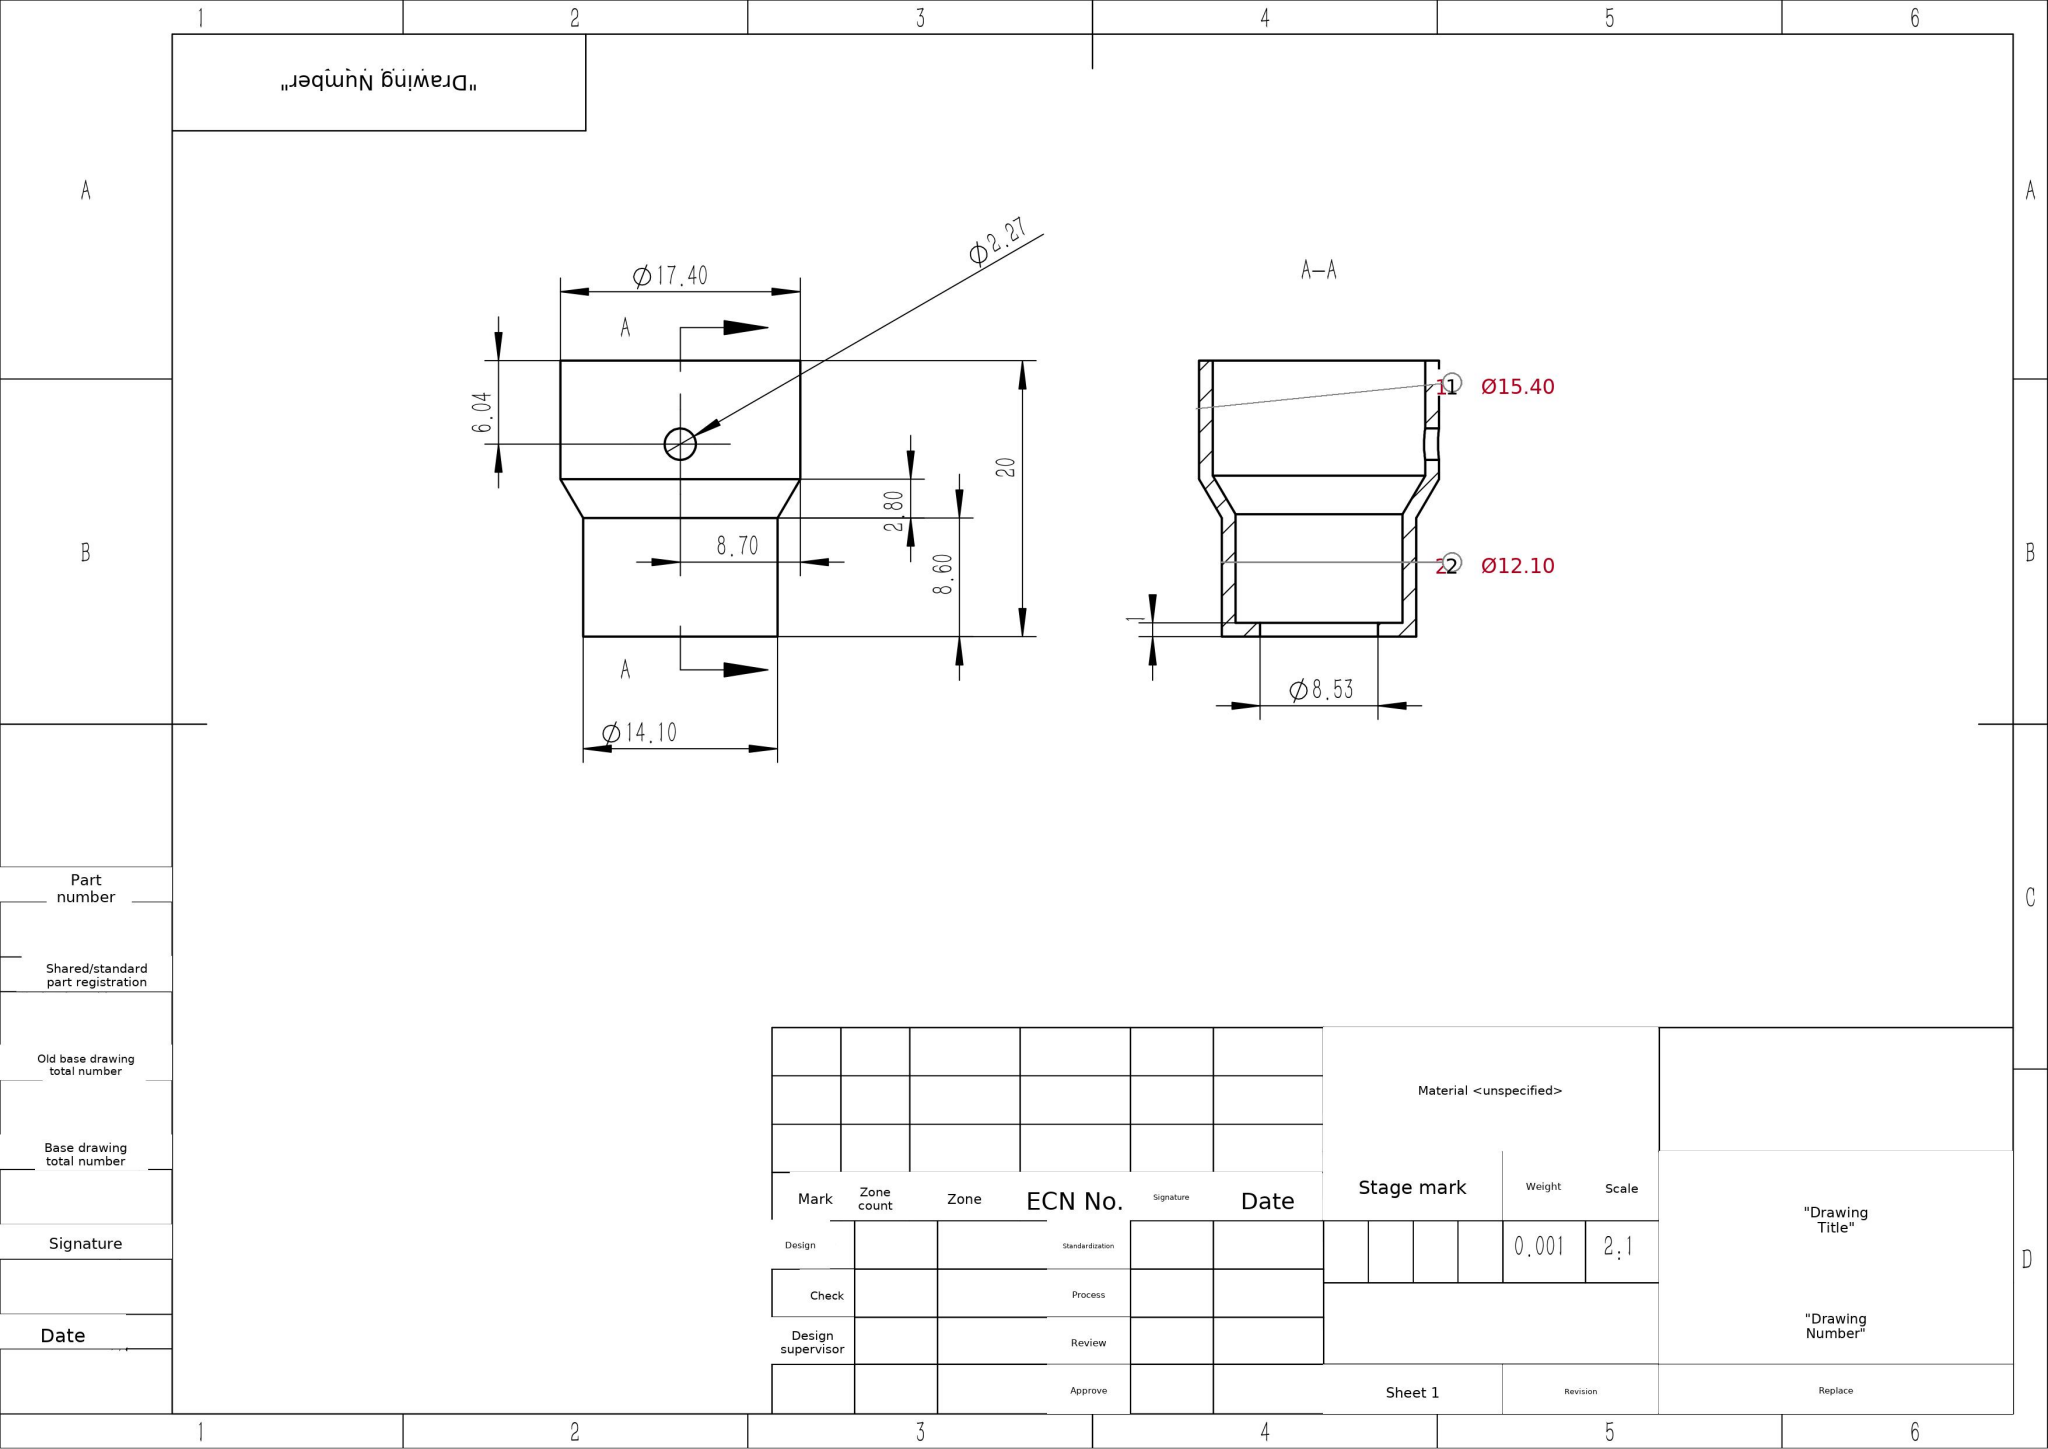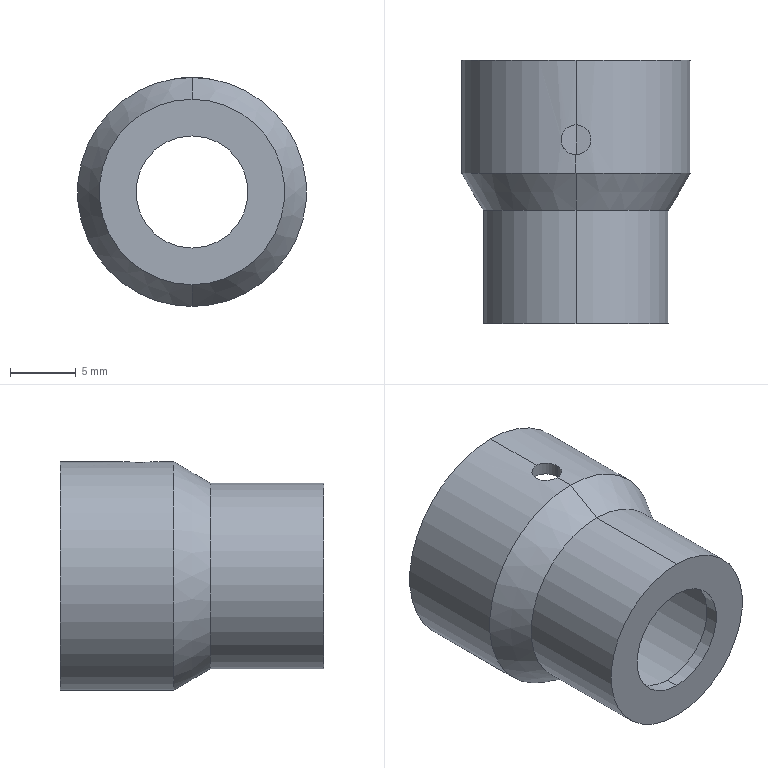Part | SolidWorks | mm | 1 solid | 19 faces | box 17.4 x 20 x 17.4 mm | volume 1000 mm3 | cylinder 12 | cone 4 | plane 3 | commonest cylinder face diameters 2.271 x2 12.1 x2 8.532 x2 14.1 x2 15.402 x2 17.402 x2
build123d program:
from build123d import *

# Parameters (mm, degrees)
SKETCH3_R          = 1.135
CUT_EXTRUDE1_DEPTH = 10


with BuildPart() as part:
    # Sketch1 → Revolve-Thin1 (revolve)
    with BuildSketch(Plane.XY, mode=Mode.PRIVATE) as revolve_thin1_sk:
        Polygon((7.701, 19), (7.701, 10.678), (6.05, 7.876), (6.05, 0), (4.266, 0), (4.266, -1), (7.05, -1), (7.05, 7.603), (8.701, 10.405), (8.701, 19), align=None)
    revolve(revolve_thin1_sk.sketch.rotate(Axis((0, 0, 0), (0, 1, 0)), 90), axis=Axis((0, 0, 0), (0, 1, 0)))

    # Sketch3 → Cut-Extrude1 (cut)
    with BuildSketch(Plane.XY):
        with Locations(Location((0, 12.957, 0), (0, 0, 180))):
            Circle(SKETCH3_R)
    extrude(amount=CUT_EXTRUDE1_DEPTH, mode=Mode.SUBTRACT)


solid = part.part
STEP:
#1=CARTESIAN_POINT('',(1.135,12.957,8.627));
#2=VERTEX_POINT('',#1);
#3=CARTESIAN_POINT('',(-0.,11.821,8.701));
#4=VERTEX_POINT('',#3);
#5=CARTESIAN_POINT('',(1.135,12.957,8.627));
#6=CARTESIAN_POINT('',(1.135,12.808,8.627));
#7=CARTESIAN_POINT('',(1.105,12.659,8.631));
#8=CARTESIAN_POINT('',(0.9922,12.385,8.644));
#9=CARTESIAN_POINT('',(0.9077,12.259,8.654));
#10=CARTESIAN_POINT('',(0.6984,12.049,8.674));
#11=CARTESIAN_POINT('',(0.5726,11.965,8.683));
#12=CARTESIAN_POINT('',(0.2976,11.851,8.697));
#13=CARTESIAN_POINT('',(0.1502,11.821,8.701));
#14=CARTESIAN_POINT('',(-0.,11.821,8.701));
#15=B_SPLINE_CURVE_WITH_KNOTS('',3,(#5,#6,#7,#8,#9,#10,#11,#12,#13,#14),.UNSPECIFIED.,.F.,.F.,(4,2,2,2,4),(0.003553,0.003998,0.004442,0.004886,0.00533),.UNSPECIFIED.);
#16=EDGE_CURVE('',#2,#4,#15,.T.);
#17=ORIENTED_EDGE('',*,*,#16,.F.);
#18=CARTESIAN_POINT('',(1.135,12.957,7.617));
#19=VERTEX_POINT('',#18);
#20=CARTESIAN_POINT('',(1.135,12.957,10.));
#21=DIRECTION('',(0.,0.,-1.));
#22=VECTOR('',#21,1000.);
#23=LINE('',#20,#22);
#24=EDGE_CURVE('',#2,#19,#23,.T.);
#25=ORIENTED_EDGE('',*,*,#24,.T.);
#26=CARTESIAN_POINT('',(0.,11.821,7.701));
#27=VERTEX_POINT('',#26);
#28=CARTESIAN_POINT('',(1.135,12.957,7.617));
#29=CARTESIAN_POINT('',(1.135,12.808,7.617));
#30=CARTESIAN_POINT('',(1.105,12.659,7.621));
#31=CARTESIAN_POINT('',(0.9922,12.385,7.637));
#32=CARTESIAN_POINT('',(0.9077,12.259,7.648));
#33=CARTESIAN_POINT('',(0.6984,12.049,7.67));
#34=CARTESIAN_POINT('',(0.5728,11.965,7.681));
#35=CARTESIAN_POINT('',(0.2976,11.851,7.696));
#36=CARTESIAN_POINT('',(0.1501,11.821,7.701));
#37=CARTESIAN_POINT('',(0.,11.821,7.701));
#38=B_SPLINE_CURVE_WITH_KNOTS('',3,(#28,#29,#30,#31,#32,#33,#34,#35,#36,#37),.UNSPECIFIED.,.F.,.F.,(4,2,2,2,4),(0.003554,0.003999,0.004443,0.004887,0.005332),.UNSPECIFIED.);
#39=EDGE_CURVE('',#19,#27,#38,.T.);
#40=ORIENTED_EDGE('',*,*,#39,.T.);
#41=CARTESIAN_POINT('',(-1.135,12.957,7.617));
#42=VERTEX_POINT('',#41);
#43=CARTESIAN_POINT('',(0.,11.821,7.701));
#44=CARTESIAN_POINT('',(-0.15,11.821,7.701));
#45=CARTESIAN_POINT('',(-0.2975,11.851,7.696));
#46=CARTESIAN_POINT('',(-0.5721,11.965,7.681));
#47=CARTESIAN_POINT('',(-0.698,12.049,7.67));
#48=CARTESIAN_POINT('',(-0.907,12.258,7.648));
#49=CARTESIAN_POINT('',(-0.9916,12.384,7.637));
#50=CARTESIAN_POINT('',(-1.105,12.657,7.622));
#51=CARTESIAN_POINT('',(-1.135,12.806,7.617));
#52=CARTESIAN_POINT('',(-1.135,12.957,7.617));
#53=B_SPLINE_CURVE_WITH_KNOTS('',3,(#43,#44,#45,#46,#47,#48,#49,#50,#51,#52),.UNSPECIFIED.,.F.,.F.,(4,2,2,2,4),(0.005332,0.005776,0.00622,0.006664,0.007108),.UNSPECIFIED.);
#54=EDGE_CURVE('',#27,#42,#53,.T.);
#55=ORIENTED_EDGE('',*,*,#54,.T.);
#56=CARTESIAN_POINT('',(-1.135,12.957,8.627));
#57=VERTEX_POINT('',#56);
#58=CARTESIAN_POINT('',(-1.135,12.957,10.));
#59=DIRECTION('',(0.,0.,-1.));
#60=VECTOR('',#59,1000.);
#61=LINE('',#58,#60);
#62=EDGE_CURVE('',#57,#42,#61,.T.);
#63=ORIENTED_EDGE('',*,*,#62,.F.);
#64=CARTESIAN_POINT('',(-0.,11.821,8.701));
#65=CARTESIAN_POINT('',(-0.15,11.821,8.701));
#66=CARTESIAN_POINT('',(-0.2974,11.851,8.697));
#67=CARTESIAN_POINT('',(-0.5721,11.965,8.683));
#68=CARTESIAN_POINT('',(-0.698,12.049,8.674));
#69=CARTESIAN_POINT('',(-0.9071,12.258,8.654));
#70=CARTESIAN_POINT('',(-0.9917,12.384,8.644));
#71=CARTESIAN_POINT('',(-1.105,12.657,8.631));
#72=CARTESIAN_POINT('',(-1.135,12.807,8.627));
#73=CARTESIAN_POINT('',(-1.135,12.957,8.627));
#74=B_SPLINE_CURVE_WITH_KNOTS('',3,(#64,#65,#66,#67,#68,#69,#70,#71,#72,#73),.UNSPECIFIED.,.F.,.F.,(4,2,2,2,4),(0.00533,0.005774,0.006218,0.006662,0.007106),.UNSPECIFIED.);
#75=EDGE_CURVE('',#4,#57,#74,.T.);
#76=ORIENTED_EDGE('',*,*,#75,.F.);
#77=EDGE_LOOP('',(#17,#25,#40,#55,#63,#76));
#78=FACE_OUTER_BOUND('',#77,.T.);
#79=CARTESIAN_POINT('',(0.,12.957,10.));
#80=DIRECTION('',(0.,0.,-1.));
#81=DIRECTION('',(-1.,0.,0.));
#82=AXIS2_PLACEMENT_3D('',#79,#80,#81);
#83=CYLINDRICAL_SURFACE('',#82,1.135);
#84=ADVANCED_FACE('',(#78),#83,.F.);
#85=CARTESIAN_POINT('',(0.,7.876,6.05));
#86=VERTEX_POINT('',#85);
#87=CARTESIAN_POINT('',(0.,7.876,-6.05));
#88=VERTEX_POINT('',#87);
#89=CARTESIAN_POINT('',(0.,7.876,0.));
#90=DIRECTION('',(0.,-1.,0.));
#91=DIRECTION('',(0.,0.,-1.));
#92=AXIS2_PLACEMENT_3D('',#89,#90,#91);
#93=CIRCLE('',#92,6.05);
#94=EDGE_CURVE('',#86,#88,#93,.T.);
#95=ORIENTED_EDGE('',*,*,#94,.T.);
#96=CARTESIAN_POINT('',(0.,10.678,-7.701));
#97=VERTEX_POINT('',#96);
#98=CARTESIAN_POINT('',(0.,7.876,-6.05));
#99=DIRECTION('',(0.,0.8616,-0.5076));
#100=VECTOR('',#99,1000.);
#101=LINE('',#98,#100);
#102=EDGE_CURVE('',#88,#97,#101,.T.);
#103=ORIENTED_EDGE('',*,*,#102,.T.);
#104=CARTESIAN_POINT('',(0.,10.678,7.701));
#105=VERTEX_POINT('',#104);
#106=CARTESIAN_POINT('',(0.,10.678,0.));
#107=DIRECTION('',(0.,-1.,0.));
#108=DIRECTION('',(0.,0.,-1.));
#109=AXIS2_PLACEMENT_3D('',#106,#107,#108);
#110=CIRCLE('',#109,7.701);
#111=EDGE_CURVE('',#105,#97,#110,.T.);
#112=ORIENTED_EDGE('',*,*,#111,.F.);
#113=CARTESIAN_POINT('',(0.,7.876,6.05));
#114=DIRECTION('',(0.,0.8616,0.5076));
#115=VECTOR('',#114,1000.);
#116=LINE('',#113,#115);
#117=EDGE_CURVE('',#86,#105,#116,.T.);
#118=ORIENTED_EDGE('',*,*,#117,.F.);
#119=EDGE_LOOP('',(#95,#103,#112,#118));
#120=FACE_OUTER_BOUND('',#119,.T.);
#121=CARTESIAN_POINT('',(0.,7.876,0.));
#122=DIRECTION('',(0.,1.,0.));
#123=DIRECTION('',(0.,0.,1.));
#124=AXIS2_PLACEMENT_3D('',#121,#122,#123);
#125=CONICAL_SURFACE('',#124,6.05,0.5324);
#126=ADVANCED_FACE('',(#120),#125,.F.);
#127=ORIENTED_EDGE('',*,*,#94,.F.);
#128=CARTESIAN_POINT('',(0.,0.,6.05));
#129=VERTEX_POINT('',#128);
#130=CARTESIAN_POINT('',(0.,0.,6.05));
#131=DIRECTION('',(0.,-1.,0.));
#132=VECTOR('',#131,1000.);
#133=LINE('',#130,#132);
#134=EDGE_CURVE('',#86,#129,#133,.T.);
#135=ORIENTED_EDGE('',*,*,#134,.T.);
#136=CARTESIAN_POINT('',(0.,0.,-6.05));
#137=VERTEX_POINT('',#136);
#138=CARTESIAN_POINT('',(0.,0.,0.));
#139=DIRECTION('',(0.,-1.,0.));
#140=DIRECTION('',(0.,0.,-1.));
#141=AXIS2_PLACEMENT_3D('',#138,#139,#140);
#142=CIRCLE('',#141,6.05);
#143=EDGE_CURVE('',#129,#137,#142,.T.);
#144=ORIENTED_EDGE('',*,*,#143,.T.);
#145=CARTESIAN_POINT('',(0.,0.,-6.05));
#146=DIRECTION('',(0.,-1.,0.));
#147=VECTOR('',#146,1000.);
#148=LINE('',#145,#147);
#149=EDGE_CURVE('',#88,#137,#148,.T.);
#150=ORIENTED_EDGE('',*,*,#149,.F.);
#151=EDGE_LOOP('',(#127,#135,#144,#150));
#152=FACE_OUTER_BOUND('',#151,.T.);
#153=CARTESIAN_POINT('',(0.,0.,0.));
#154=DIRECTION('',(0.,-1.,0.));
#155=DIRECTION('',(0.,0.,-1.));
#156=AXIS2_PLACEMENT_3D('',#153,#154,#155);
#157=CYLINDRICAL_SURFACE('',#156,6.05);
#158=ADVANCED_FACE('',(#152),#157,.F.);
#159=CARTESIAN_POINT('',(0.,0.,4.266));
#160=VERTEX_POINT('',#159);
#161=CARTESIAN_POINT('',(0.,0.,-4.266));
#162=VERTEX_POINT('',#161);
#163=CARTESIAN_POINT('',(0.,0.,0.));
#164=DIRECTION('',(0.,-1.,0.));
#165=DIRECTION('',(0.,0.,-1.));
#166=AXIS2_PLACEMENT_3D('',#163,#164,#165);
#167=CIRCLE('',#166,4.266);
#168=EDGE_CURVE('',#160,#162,#167,.T.);
#169=ORIENTED_EDGE('',*,*,#168,.F.);
#170=CARTESIAN_POINT('',(0.,-1.,4.266));
#171=VERTEX_POINT('',#170);
#172=CARTESIAN_POINT('',(0.,0.,4.266));
#173=DIRECTION('',(0.,-1.,0.));
#174=VECTOR('',#173,1000.);
#175=LINE('',#172,#174);
#176=EDGE_CURVE('',#160,#171,#175,.T.);
#177=ORIENTED_EDGE('',*,*,#176,.T.);
#178=CARTESIAN_POINT('',(0.,-1.,-4.266));
#179=VERTEX_POINT('',#178);
#180=CARTESIAN_POINT('',(0.,-1.,0.));
#181=DIRECTION('',(0.,-1.,0.));
#182=DIRECTION('',(0.,0.,-1.));
#183=AXIS2_PLACEMENT_3D('',#180,#181,#182);
#184=CIRCLE('',#183,4.266);
#185=EDGE_CURVE('',#171,#179,#184,.T.);
#186=ORIENTED_EDGE('',*,*,#185,.T.);
#187=CARTESIAN_POINT('',(0.,0.,-4.266));
#188=DIRECTION('',(0.,-1.,0.));
#189=VECTOR('',#188,1000.);
#190=LINE('',#187,#189);
#191=EDGE_CURVE('',#162,#179,#190,.T.);
#192=ORIENTED_EDGE('',*,*,#191,.F.);
#193=EDGE_LOOP('',(#169,#177,#186,#192));
#194=FACE_OUTER_BOUND('',#193,.T.);
#195=CARTESIAN_POINT('',(0.,0.,0.));
#196=DIRECTION('',(0.,-1.,0.));
#197=DIRECTION('',(0.,0.,-1.));
#198=AXIS2_PLACEMENT_3D('',#195,#196,#197);
#199=CYLINDRICAL_SURFACE('',#198,4.266);
#200=ADVANCED_FACE('',(#194),#199,.F.);
#201=CARTESIAN_POINT('',(0.,7.603,-7.05));
#202=VERTEX_POINT('',#201);
#203=CARTESIAN_POINT('',(0.,7.603,7.05));
#204=VERTEX_POINT('',#203);
#205=CARTESIAN_POINT('',(0.,7.603,0.));
#206=DIRECTION('',(0.,-1.,0.));
#207=DIRECTION('',(0.,0.,-1.));
#208=AXIS2_PLACEMENT_3D('',#205,#206,#207);
#209=CIRCLE('',#208,7.05);
#210=EDGE_CURVE('',#202,#204,#209,.T.);
#211=ORIENTED_EDGE('',*,*,#210,.T.);
#212=CARTESIAN_POINT('',(0.,-1.,7.05));
#213=VERTEX_POINT('',#212);
#214=CARTESIAN_POINT('',(0.,0.,7.05));
#215=DIRECTION('',(0.,-1.,0.));
#216=VECTOR('',#215,1000.);
#217=LINE('',#214,#216);
#218=EDGE_CURVE('',#204,#213,#217,.T.);
#219=ORIENTED_EDGE('',*,*,#218,.T.);
#220=CARTESIAN_POINT('',(0.,-1.,-7.05));
#221=VERTEX_POINT('',#220);
#222=CARTESIAN_POINT('',(0.,-1.,0.));
#223=DIRECTION('',(0.,-1.,0.));
#224=DIRECTION('',(0.,0.,-1.));
#225=AXIS2_PLACEMENT_3D('',#222,#223,#224);
#226=CIRCLE('',#225,7.05);
#227=EDGE_CURVE('',#221,#213,#226,.T.);
#228=ORIENTED_EDGE('',*,*,#227,.F.);
#229=CARTESIAN_POINT('',(0.,0.,-7.05));
#230=DIRECTION('',(0.,-1.,0.));
#231=VECTOR('',#230,1000.);
#232=LINE('',#229,#231);
#233=EDGE_CURVE('',#202,#221,#232,.T.);
#234=ORIENTED_EDGE('',*,*,#233,.F.);
#235=EDGE_LOOP('',(#211,#219,#228,#234));
#236=FACE_OUTER_BOUND('',#235,.T.);
#237=CARTESIAN_POINT('',(0.,0.,0.));
#238=DIRECTION('',(0.,-1.,0.));
#239=DIRECTION('',(0.,0.,-1.));
#240=AXIS2_PLACEMENT_3D('',#237,#238,#239);
#241=CYLINDRICAL_SURFACE('',#240,7.05);
#242=ADVANCED_FACE('',(#236),#241,.T.);
#243=ORIENTED_EDGE('',*,*,#210,.F.);
#244=CARTESIAN_POINT('',(0.,10.405,-8.701));
#245=VERTEX_POINT('',#244);
#246=CARTESIAN_POINT('',(0.,7.603,-7.05));
#247=DIRECTION('',(0.,0.8616,-0.5076));
#248=VECTOR('',#247,1000.);
#249=LINE('',#246,#248);
#250=EDGE_CURVE('',#202,#245,#249,.T.);
#251=ORIENTED_EDGE('',*,*,#250,.T.);
#252=CARTESIAN_POINT('',(0.,10.405,8.701));
#253=VERTEX_POINT('',#252);
#254=CARTESIAN_POINT('',(0.,10.405,0.));
#255=DIRECTION('',(0.,-1.,0.));
#256=DIRECTION('',(0.,0.,-1.));
#257=AXIS2_PLACEMENT_3D('',#254,#255,#256);
#258=CIRCLE('',#257,8.701);
#259=EDGE_CURVE('',#245,#253,#258,.T.);
#260=ORIENTED_EDGE('',*,*,#259,.T.);
#261=CARTESIAN_POINT('',(0.,7.603,7.05));
#262=DIRECTION('',(0.,0.8616,0.5076));
#263=VECTOR('',#262,1000.);
#264=LINE('',#261,#263);
#265=EDGE_CURVE('',#204,#253,#264,.T.);
#266=ORIENTED_EDGE('',*,*,#265,.F.);
#267=EDGE_LOOP('',(#243,#251,#260,#266));
#268=FACE_OUTER_BOUND('',#267,.T.);
#269=CARTESIAN_POINT('',(0.,7.603,0.));
#270=DIRECTION('',(0.,1.,0.));
#271=DIRECTION('',(0.,0.,1.));
#272=AXIS2_PLACEMENT_3D('',#269,#270,#271);
#273=CONICAL_SURFACE('',#272,7.05,0.5324);
#274=ADVANCED_FACE('',(#268),#273,.T.);
#275=CARTESIAN_POINT('',(0.,19.,7.701));
#276=VERTEX_POINT('',#275);
#277=CARTESIAN_POINT('',(0.,19.,-7.701));
#278=VERTEX_POINT('',#277);
#279=CARTESIAN_POINT('',(0.,19.,0.));
#280=DIRECTION('',(0.,-1.,0.));
#281=DIRECTION('',(0.,0.,-1.));
#282=AXIS2_PLACEMENT_3D('',#279,#280,#281);
#283=CIRCLE('',#282,7.701);
#284=EDGE_CURVE('',#276,#278,#283,.T.);
#285=ORIENTED_EDGE('',*,*,#284,.F.);
#286=CARTESIAN_POINT('',(0.,14.092,7.701));
#287=VERTEX_POINT('',#286);
#288=CARTESIAN_POINT('',(0.,0.,7.701));
#289=DIRECTION('',(0.,-1.,0.));
#290=VECTOR('',#289,1000.);
#291=LINE('',#288,#290);
#292=EDGE_CURVE('',#276,#287,#291,.T.);
#293=ORIENTED_EDGE('',*,*,#292,.T.);
#294=CARTESIAN_POINT('',(-1.135,12.957,7.617));
#295=CARTESIAN_POINT('',(-1.135,13.107,7.617));
#296=CARTESIAN_POINT('',(-1.106,13.254,7.621));
#297=CARTESIAN_POINT('',(-0.9915,13.529,7.637));
#298=CARTESIAN_POINT('',(-0.9071,13.655,7.648));
#299=CARTESIAN_POINT('',(-0.6978,13.864,7.67));
#300=CARTESIAN_POINT('',(-0.5712,13.949,7.681));
#301=CARTESIAN_POINT('',(-0.298,14.062,7.696));
#302=CARTESIAN_POINT('',(-0.1484,14.092,7.701));
#303=CARTESIAN_POINT('',(0.,14.092,7.701));
#304=B_SPLINE_CURVE_WITH_KNOTS('',3,(#294,#295,#296,#297,#298,#299,#300,#301,#302,#303),.UNSPECIFIED.,.F.,.F.,(4,2,2,2,4),(0.,0.0004444,0.0008888,0.001333,0.001778),.UNSPECIFIED.);
#305=EDGE_CURVE('',#42,#287,#304,.T.);
#306=ORIENTED_EDGE('',*,*,#305,.F.);
#307=ORIENTED_EDGE('',*,*,#54,.F.);
#308=CARTESIAN_POINT('',(0.,0.,7.701));
#309=DIRECTION('',(0.,-1.,0.));
#310=VECTOR('',#309,1000.);
#311=LINE('',#308,#310);
#312=EDGE_CURVE('',#27,#105,#311,.T.);
#313=ORIENTED_EDGE('',*,*,#312,.T.);
#314=ORIENTED_EDGE('',*,*,#111,.T.);
#315=CARTESIAN_POINT('',(0.,0.,-7.701));
#316=DIRECTION('',(0.,-1.,0.));
#317=VECTOR('',#316,1000.);
#318=LINE('',#315,#317);
#319=EDGE_CURVE('',#278,#97,#318,.T.);
#320=ORIENTED_EDGE('',*,*,#319,.F.);
#321=EDGE_LOOP('',(#285,#293,#306,#307,#313,#314,#320));
#322=FACE_OUTER_BOUND('',#321,.T.);
#323=CARTESIAN_POINT('',(0.,0.,0.));
#324=DIRECTION('',(0.,-1.,0.));
#325=DIRECTION('',(0.,0.,-1.));
#326=AXIS2_PLACEMENT_3D('',#323,#324,#325);
#327=CYLINDRICAL_SURFACE('',#326,7.701);
#328=ADVANCED_FACE('',(#322),#327,.F.);
#329=CARTESIAN_POINT('',(0.,19.,-8.701));
#330=VERTEX_POINT('',#329);
#331=CARTESIAN_POINT('',(0.,19.,8.701));
#332=VERTEX_POINT('',#331);
#333=CARTESIAN_POINT('',(0.,19.,0.));
#334=DIRECTION('',(0.,-1.,0.));
#335=DIRECTION('',(0.,0.,-1.));
#336=AXIS2_PLACEMENT_3D('',#333,#334,#335);
#337=CIRCLE('',#336,8.701);
#338=EDGE_CURVE('',#330,#332,#337,.T.);
#339=ORIENTED_EDGE('',*,*,#338,.T.);
#340=CARTESIAN_POINT('',(0.,14.092,8.701));
#341=VERTEX_POINT('',#340);
#342=CARTESIAN_POINT('',(0.,0.,8.701));
#343=DIRECTION('',(0.,-1.,0.));
#344=VECTOR('',#343,1000.);
#345=LINE('',#342,#344);
#346=EDGE_CURVE('',#332,#341,#345,.T.);
#347=ORIENTED_EDGE('',*,*,#346,.T.);
#348=CARTESIAN_POINT('',(0.,14.092,8.701));
#349=CARTESIAN_POINT('',(0.1482,14.092,8.701));
#350=CARTESIAN_POINT('',(0.2971,14.062,8.697));
#351=CARTESIAN_POINT('',(0.5721,13.948,8.683));
#352=CARTESIAN_POINT('',(0.697,13.865,8.674));
#353=CARTESIAN_POINT('',(0.9087,13.653,8.654));
#354=CARTESIAN_POINT('',(0.992,13.529,8.644));
#355=CARTESIAN_POINT('',(1.106,13.254,8.631));
#356=CARTESIAN_POINT('',(1.135,13.105,8.627));
#357=CARTESIAN_POINT('',(1.135,12.957,8.627));
#358=B_SPLINE_CURVE_WITH_KNOTS('',3,(#348,#349,#350,#351,#352,#353,#354,#355,#356,#357),.UNSPECIFIED.,.F.,.F.,(4,2,2,2,4),(0.001777,0.002221,0.002665,0.003109,0.003553),.UNSPECIFIED.);
#359=EDGE_CURVE('',#341,#2,#358,.T.);
#360=ORIENTED_EDGE('',*,*,#359,.T.);
#361=ORIENTED_EDGE('',*,*,#16,.T.);
#362=CARTESIAN_POINT('',(0.,0.,8.701));
#363=DIRECTION('',(0.,-1.,0.));
#364=VECTOR('',#363,1000.);
#365=LINE('',#362,#364);
#366=EDGE_CURVE('',#4,#253,#365,.T.);
#367=ORIENTED_EDGE('',*,*,#366,.T.);
#368=ORIENTED_EDGE('',*,*,#259,.F.);
#369=CARTESIAN_POINT('',(0.,0.,-8.701));
#370=DIRECTION('',(0.,-1.,0.));
#371=VECTOR('',#370,1000.);
#372=LINE('',#369,#371);
#373=EDGE_CURVE('',#330,#245,#372,.T.);
#374=ORIENTED_EDGE('',*,*,#373,.F.);
#375=EDGE_LOOP('',(#339,#347,#360,#361,#367,#368,#374));
#376=FACE_OUTER_BOUND('',#375,.T.);
#377=CARTESIAN_POINT('',(0.,0.,0.));
#378=DIRECTION('',(0.,-1.,0.));
#379=DIRECTION('',(0.,0.,-1.));
#380=AXIS2_PLACEMENT_3D('',#377,#378,#379);
#381=CYLINDRICAL_SURFACE('',#380,8.701);
#382=ADVANCED_FACE('',(#376),#381,.T.);
#383=ORIENTED_EDGE('',*,*,#346,.F.);
#384=CARTESIAN_POINT('',(0.,19.,0.));
#385=DIRECTION('',(0.,-1.,0.));
#386=DIRECTION('',(0.,0.,-1.));
#387=AXIS2_PLACEMENT_3D('',#384,#385,#386);
#388=CIRCLE('',#387,8.701);
#389=EDGE_CURVE('',#332,#330,#388,.T.);
#390=ORIENTED_EDGE('',*,*,#389,.T.);
#391=ORIENTED_EDGE('',*,*,#373,.T.);
#392=CARTESIAN_POINT('',(0.,10.405,0.));
#393=DIRECTION('',(0.,-1.,0.));
#394=DIRECTION('',(0.,0.,-1.));
#395=AXIS2_PLACEMENT_3D('',#392,#393,#394);
#396=CIRCLE('',#395,8.701);
#397=EDGE_CURVE('',#253,#245,#396,.T.);
#398=ORIENTED_EDGE('',*,*,#397,.F.);
#399=ORIENTED_EDGE('',*,*,#366,.F.);
#400=ORIENTED_EDGE('',*,*,#75,.T.);
#401=CARTESIAN_POINT('',(-1.135,12.957,8.627));
#402=CARTESIAN_POINT('',(-1.135,13.107,8.627));
#403=CARTESIAN_POINT('',(-1.106,13.254,8.631));
#404=CARTESIAN_POINT('',(-0.9916,13.529,8.644));
#405=CARTESIAN_POINT('',(-0.9072,13.655,8.654));
#406=CARTESIAN_POINT('',(-0.6978,13.864,8.674));
#407=CARTESIAN_POINT('',(-0.5712,13.949,8.683));
#408=CARTESIAN_POINT('',(-0.2979,14.062,8.697));
#409=CARTESIAN_POINT('',(-0.1483,14.092,8.701));
#410=CARTESIAN_POINT('',(0.,14.092,8.701));
#411=B_SPLINE_CURVE_WITH_KNOTS('',3,(#401,#402,#403,#404,#405,#406,#407,#408,#409,#410),.UNSPECIFIED.,.F.,.F.,(4,2,2,2,4),(0.,0.0004443,0.0008885,0.001333,0.001777),.UNSPECIFIED.);
#412=EDGE_CURVE('',#57,#341,#411,.T.);
#413=ORIENTED_EDGE('',*,*,#412,.T.);
#414=EDGE_LOOP('',(#383,#390,#391,#398,#399,#400,#413));
#415=FACE_OUTER_BOUND('',#414,.T.);
#416=CARTESIAN_POINT('',(0.,0.,0.));
#417=DIRECTION('',(0.,-1.,0.));
#418=DIRECTION('',(0.,0.,-1.));
#419=AXIS2_PLACEMENT_3D('',#416,#417,#418);
#420=CYLINDRICAL_SURFACE('',#419,8.701);
#421=ADVANCED_FACE('',(#415),#420,.T.);
#422=ORIENTED_EDGE('',*,*,#292,.F.);
#423=CARTESIAN_POINT('',(0.,19.,0.));
#424=DIRECTION('',(0.,-1.,0.));
#425=DIRECTION('',(0.,0.,-1.));
#426=AXIS2_PLACEMENT_3D('',#423,#424,#425);
#427=CIRCLE('',#426,7.701);
#428=EDGE_CURVE('',#278,#276,#427,.T.);
#429=ORIENTED_EDGE('',*,*,#428,.F.);
#430=ORIENTED_EDGE('',*,*,#319,.T.);
#431=CARTESIAN_POINT('',(0.,10.678,0.));
#432=DIRECTION('',(0.,-1.,0.));
#433=DIRECTION('',(0.,0.,-1.));
#434=AXIS2_PLACEMENT_3D('',#431,#432,#433);
#435=CIRCLE('',#434,7.701);
#436=EDGE_CURVE('',#97,#105,#435,.T.);
#437=ORIENTED_EDGE('',*,*,#436,.T.);
#438=ORIENTED_EDGE('',*,*,#312,.F.);
#439=ORIENTED_EDGE('',*,*,#39,.F.);
#440=CARTESIAN_POINT('',(0.,14.092,7.701));
#441=CARTESIAN_POINT('',(0.1483,14.092,7.701));
#442=CARTESIAN_POINT('',(0.2971,14.062,7.696));
#443=CARTESIAN_POINT('',(0.5722,13.948,7.681));
#444=CARTESIAN_POINT('',(0.6971,13.865,7.67));
#445=CARTESIAN_POINT('',(0.9087,13.653,7.648));
#446=CARTESIAN_POINT('',(0.9919,13.529,7.637));
#447=CARTESIAN_POINT('',(1.106,13.254,7.621));
#448=CARTESIAN_POINT('',(1.135,13.105,7.617));
#449=CARTESIAN_POINT('',(1.135,12.957,7.617));
#450=B_SPLINE_CURVE_WITH_KNOTS('',3,(#440,#441,#442,#443,#444,#445,#446,#447,#448,#449),.UNSPECIFIED.,.F.,.F.,(4,2,2,2,4),(0.001778,0.002222,0.002666,0.00311,0.003554),.UNSPECIFIED.);
#451=EDGE_CURVE('',#287,#19,#450,.T.);
#452=ORIENTED_EDGE('',*,*,#451,.F.);
#453=EDGE_LOOP('',(#422,#429,#430,#437,#438,#439,#452));
#454=FACE_OUTER_BOUND('',#453,.T.);
#455=CARTESIAN_POINT('',(0.,0.,0.));
#456=DIRECTION('',(0.,-1.,0.));
#457=DIRECTION('',(0.,0.,-1.));
#458=AXIS2_PLACEMENT_3D('',#455,#456,#457);
#459=CYLINDRICAL_SURFACE('',#458,7.701);
#460=ADVANCED_FACE('',(#454),#459,.F.);
#461=ORIENTED_EDGE('',*,*,#250,.F.);
#462=CARTESIAN_POINT('',(0.,7.603,0.));
#463=DIRECTION('',(0.,-1.,0.));
#464=DIRECTION('',(0.,0.,-1.));
#465=AXIS2_PLACEMENT_3D('',#462,#463,#464);
#466=CIRCLE('',#465,7.05);
#467=EDGE_CURVE('',#204,#202,#466,.T.);
#468=ORIENTED_EDGE('',*,*,#467,.F.);
#469=ORIENTED_EDGE('',*,*,#265,.T.);
#470=ORIENTED_EDGE('',*,*,#397,.T.);
#471=EDGE_LOOP('',(#461,#468,#469,#470));
#472=FACE_OUTER_BOUND('',#471,.T.);
#473=CARTESIAN_POINT('',(0.,7.603,0.));
#474=DIRECTION('',(0.,1.,0.));
#475=DIRECTION('',(0.,0.,1.));
#476=AXIS2_PLACEMENT_3D('',#473,#474,#475);
#477=CONICAL_SURFACE('',#476,7.05,0.5324);
#478=ADVANCED_FACE('',(#472),#477,.T.);
#479=ORIENTED_EDGE('',*,*,#218,.F.);
#480=ORIENTED_EDGE('',*,*,#467,.T.);
#481=ORIENTED_EDGE('',*,*,#233,.T.);
#482=CARTESIAN_POINT('',(0.,-1.,0.));
#483=DIRECTION('',(0.,-1.,0.));
#484=DIRECTION('',(0.,0.,-1.));
#485=AXIS2_PLACEMENT_3D('',#482,#483,#484);
#486=CIRCLE('',#485,7.05);
#487=EDGE_CURVE('',#213,#221,#486,.T.);
#488=ORIENTED_EDGE('',*,*,#487,.F.);
#489=EDGE_LOOP('',(#479,#480,#481,#488));
#490=FACE_OUTER_BOUND('',#489,.T.);
#491=CARTESIAN_POINT('',(0.,0.,0.));
#492=DIRECTION('',(0.,-1.,0.));
#493=DIRECTION('',(0.,0.,-1.));
#494=AXIS2_PLACEMENT_3D('',#491,#492,#493);
#495=CYLINDRICAL_SURFACE('',#494,7.05);
#496=ADVANCED_FACE('',(#490),#495,.T.);
#497=ORIENTED_EDGE('',*,*,#227,.T.);
#498=ORIENTED_EDGE('',*,*,#487,.T.);
#499=EDGE_LOOP('',(#497,#498));
#500=FACE_OUTER_BOUND('',#499,.T.);
#501=CARTESIAN_POINT('',(0.,-1.,0.));
#502=DIRECTION('',(0.,-1.,0.));
#503=DIRECTION('',(0.,0.,-1.));
#504=AXIS2_PLACEMENT_3D('',#501,#502,#503);
#505=CIRCLE('',#504,4.266);
#506=EDGE_CURVE('',#179,#171,#505,.T.);
#507=ORIENTED_EDGE('',*,*,#506,.F.);
#508=ORIENTED_EDGE('',*,*,#185,.F.);
#509=EDGE_LOOP('',(#507,#508));
#510=FACE_BOUND('',#509,.T.);
#511=CARTESIAN_POINT('',(6.05,-1.,0.));
#512=DIRECTION('',(0.,-1.,0.));
#513=DIRECTION('',(0.,0.,-1.));
#514=AXIS2_PLACEMENT_3D('',#511,#512,#513);
#515=PLANE('',#514);
#516=ADVANCED_FACE('',(#500,#510),#515,.T.);
#517=ORIENTED_EDGE('',*,*,#176,.F.);
#518=CARTESIAN_POINT('',(0.,0.,0.));
#519=DIRECTION('',(0.,-1.,0.));
#520=DIRECTION('',(0.,0.,-1.));
#521=AXIS2_PLACEMENT_3D('',#518,#519,#520);
#522=CIRCLE('',#521,4.266);
#523=EDGE_CURVE('',#162,#160,#522,.T.);
#524=ORIENTED_EDGE('',*,*,#523,.F.);
#525=ORIENTED_EDGE('',*,*,#191,.T.);
#526=ORIENTED_EDGE('',*,*,#506,.T.);
#527=EDGE_LOOP('',(#517,#524,#525,#526));
#528=FACE_OUTER_BOUND('',#527,.T.);
#529=CARTESIAN_POINT('',(0.,0.,0.));
#530=DIRECTION('',(0.,-1.,0.));
#531=DIRECTION('',(0.,0.,-1.));
#532=AXIS2_PLACEMENT_3D('',#529,#530,#531);
#533=CYLINDRICAL_SURFACE('',#532,4.266);
#534=ADVANCED_FACE('',(#528),#533,.F.);
#535=CARTESIAN_POINT('',(0.,0.,0.));
#536=DIRECTION('',(0.,-1.,0.));
#537=DIRECTION('',(0.,0.,-1.));
#538=AXIS2_PLACEMENT_3D('',#535,#536,#537);
#539=CIRCLE('',#538,6.05);
#540=EDGE_CURVE('',#137,#129,#539,.T.);
#541=ORIENTED_EDGE('',*,*,#540,.F.);
#542=ORIENTED_EDGE('',*,*,#143,.F.);
#543=EDGE_LOOP('',(#541,#542));
#544=FACE_OUTER_BOUND('',#543,.T.);
#545=ORIENTED_EDGE('',*,*,#523,.T.);
#546=ORIENTED_EDGE('',*,*,#168,.T.);
#547=EDGE_LOOP('',(#545,#546));
#548=FACE_BOUND('',#547,.T.);
#549=CARTESIAN_POINT('',(6.05,0.,0.));
#550=DIRECTION('',(0.,-1.,0.));
#551=DIRECTION('',(0.,0.,-1.));
#552=AXIS2_PLACEMENT_3D('',#549,#550,#551);
#553=PLANE('',#552);
#554=ADVANCED_FACE('',(#544,#548),#553,.F.);
#555=ORIENTED_EDGE('',*,*,#134,.F.);
#556=CARTESIAN_POINT('',(0.,7.876,0.));
#557=DIRECTION('',(0.,-1.,0.));
#558=DIRECTION('',(0.,0.,-1.));
#559=AXIS2_PLACEMENT_3D('',#556,#557,#558);
#560=CIRCLE('',#559,6.05);
#561=EDGE_CURVE('',#88,#86,#560,.T.);
#562=ORIENTED_EDGE('',*,*,#561,.F.);
#563=ORIENTED_EDGE('',*,*,#149,.T.);
#564=ORIENTED_EDGE('',*,*,#540,.T.);
#565=EDGE_LOOP('',(#555,#562,#563,#564));
#566=FACE_OUTER_BOUND('',#565,.T.);
#567=CARTESIAN_POINT('',(0.,0.,0.));
#568=DIRECTION('',(0.,-1.,0.));
#569=DIRECTION('',(0.,0.,-1.));
#570=AXIS2_PLACEMENT_3D('',#567,#568,#569);
#571=CYLINDRICAL_SURFACE('',#570,6.05);
#572=ADVANCED_FACE('',(#566),#571,.F.);
#573=ORIENTED_EDGE('',*,*,#102,.F.);
#574=ORIENTED_EDGE('',*,*,#561,.T.);
#575=ORIENTED_EDGE('',*,*,#117,.T.);
#576=ORIENTED_EDGE('',*,*,#436,.F.);
#577=EDGE_LOOP('',(#573,#574,#575,#576));
#578=FACE_OUTER_BOUND('',#577,.T.);
#579=CARTESIAN_POINT('',(0.,7.876,0.));
#580=DIRECTION('',(0.,1.,0.));
#581=DIRECTION('',(0.,0.,1.));
#582=AXIS2_PLACEMENT_3D('',#579,#580,#581);
#583=CONICAL_SURFACE('',#582,6.05,0.5324);
#584=ADVANCED_FACE('',(#578),#583,.F.);
#585=ORIENTED_EDGE('',*,*,#338,.F.);
#586=ORIENTED_EDGE('',*,*,#389,.F.);
#587=EDGE_LOOP('',(#585,#586));
#588=FACE_OUTER_BOUND('',#587,.T.);
#589=ORIENTED_EDGE('',*,*,#428,.T.);
#590=ORIENTED_EDGE('',*,*,#284,.T.);
#591=EDGE_LOOP('',(#589,#590));
#592=FACE_BOUND('',#591,.T.);
#593=CARTESIAN_POINT('',(7.701,19.,0.));
#594=DIRECTION('',(0.,-1.,0.));
#595=DIRECTION('',(0.,0.,-1.));
#596=AXIS2_PLACEMENT_3D('',#593,#594,#595);
#597=PLANE('',#596);
#598=ADVANCED_FACE('',(#588,#592),#597,.F.);
#599=ORIENTED_EDGE('',*,*,#24,.F.);
#600=ORIENTED_EDGE('',*,*,#359,.F.);
#601=ORIENTED_EDGE('',*,*,#412,.F.);
#602=ORIENTED_EDGE('',*,*,#62,.T.);
#603=ORIENTED_EDGE('',*,*,#305,.T.);
#604=ORIENTED_EDGE('',*,*,#451,.T.);
#605=EDGE_LOOP('',(#599,#600,#601,#602,#603,#604));
#606=FACE_OUTER_BOUND('',#605,.T.);
#607=CARTESIAN_POINT('',(0.,12.957,10.));
#608=DIRECTION('',(0.,0.,-1.));
#609=DIRECTION('',(-1.,0.,0.));
#610=AXIS2_PLACEMENT_3D('',#607,#608,#609);
#611=CYLINDRICAL_SURFACE('',#610,1.135);
#612=ADVANCED_FACE('',(#606),#611,.F.);
#613=CLOSED_SHELL('',(#84,#126,#158,#200,#242,#274,#328,#382,#421,#460,#478,#496,#516,#534,#554,#572,#584,#598,#612));
#614=MANIFOLD_SOLID_BREP('',#613);
#615=CARTESIAN_POINT('',(0.,0.,0.));
#616=DIRECTION('',(0.,0.,1.));
#617=DIRECTION('',(1.,0.,0.));
#618=AXIS2_PLACEMENT_3D('',#615,#616,#617);
#619=(LENGTH_UNIT()NAMED_UNIT(*)SI_UNIT(.MILLI.,.METRE.));
#620=UNCERTAINTY_MEASURE_WITH_UNIT(LENGTH_MEASURE(0.00001),#619,'','');
#621=(NAMED_UNIT(*)PLANE_ANGLE_UNIT()SI_UNIT($,.RADIAN.));
#622=(NAMED_UNIT(*)SI_UNIT($,.STERADIAN.)SOLID_ANGLE_UNIT());
#623=(GEOMETRIC_REPRESENTATION_CONTEXT(3)GLOBAL_UNCERTAINTY_ASSIGNED_CONTEXT((#620))GLOBAL_UNIT_ASSIGNED_CONTEXT((#619,#621,#622))REPRESENTATION_CONTEXT('',''));
#624=ADVANCED_BREP_SHAPE_REPRESENTATION('',(#614,#618),#623);